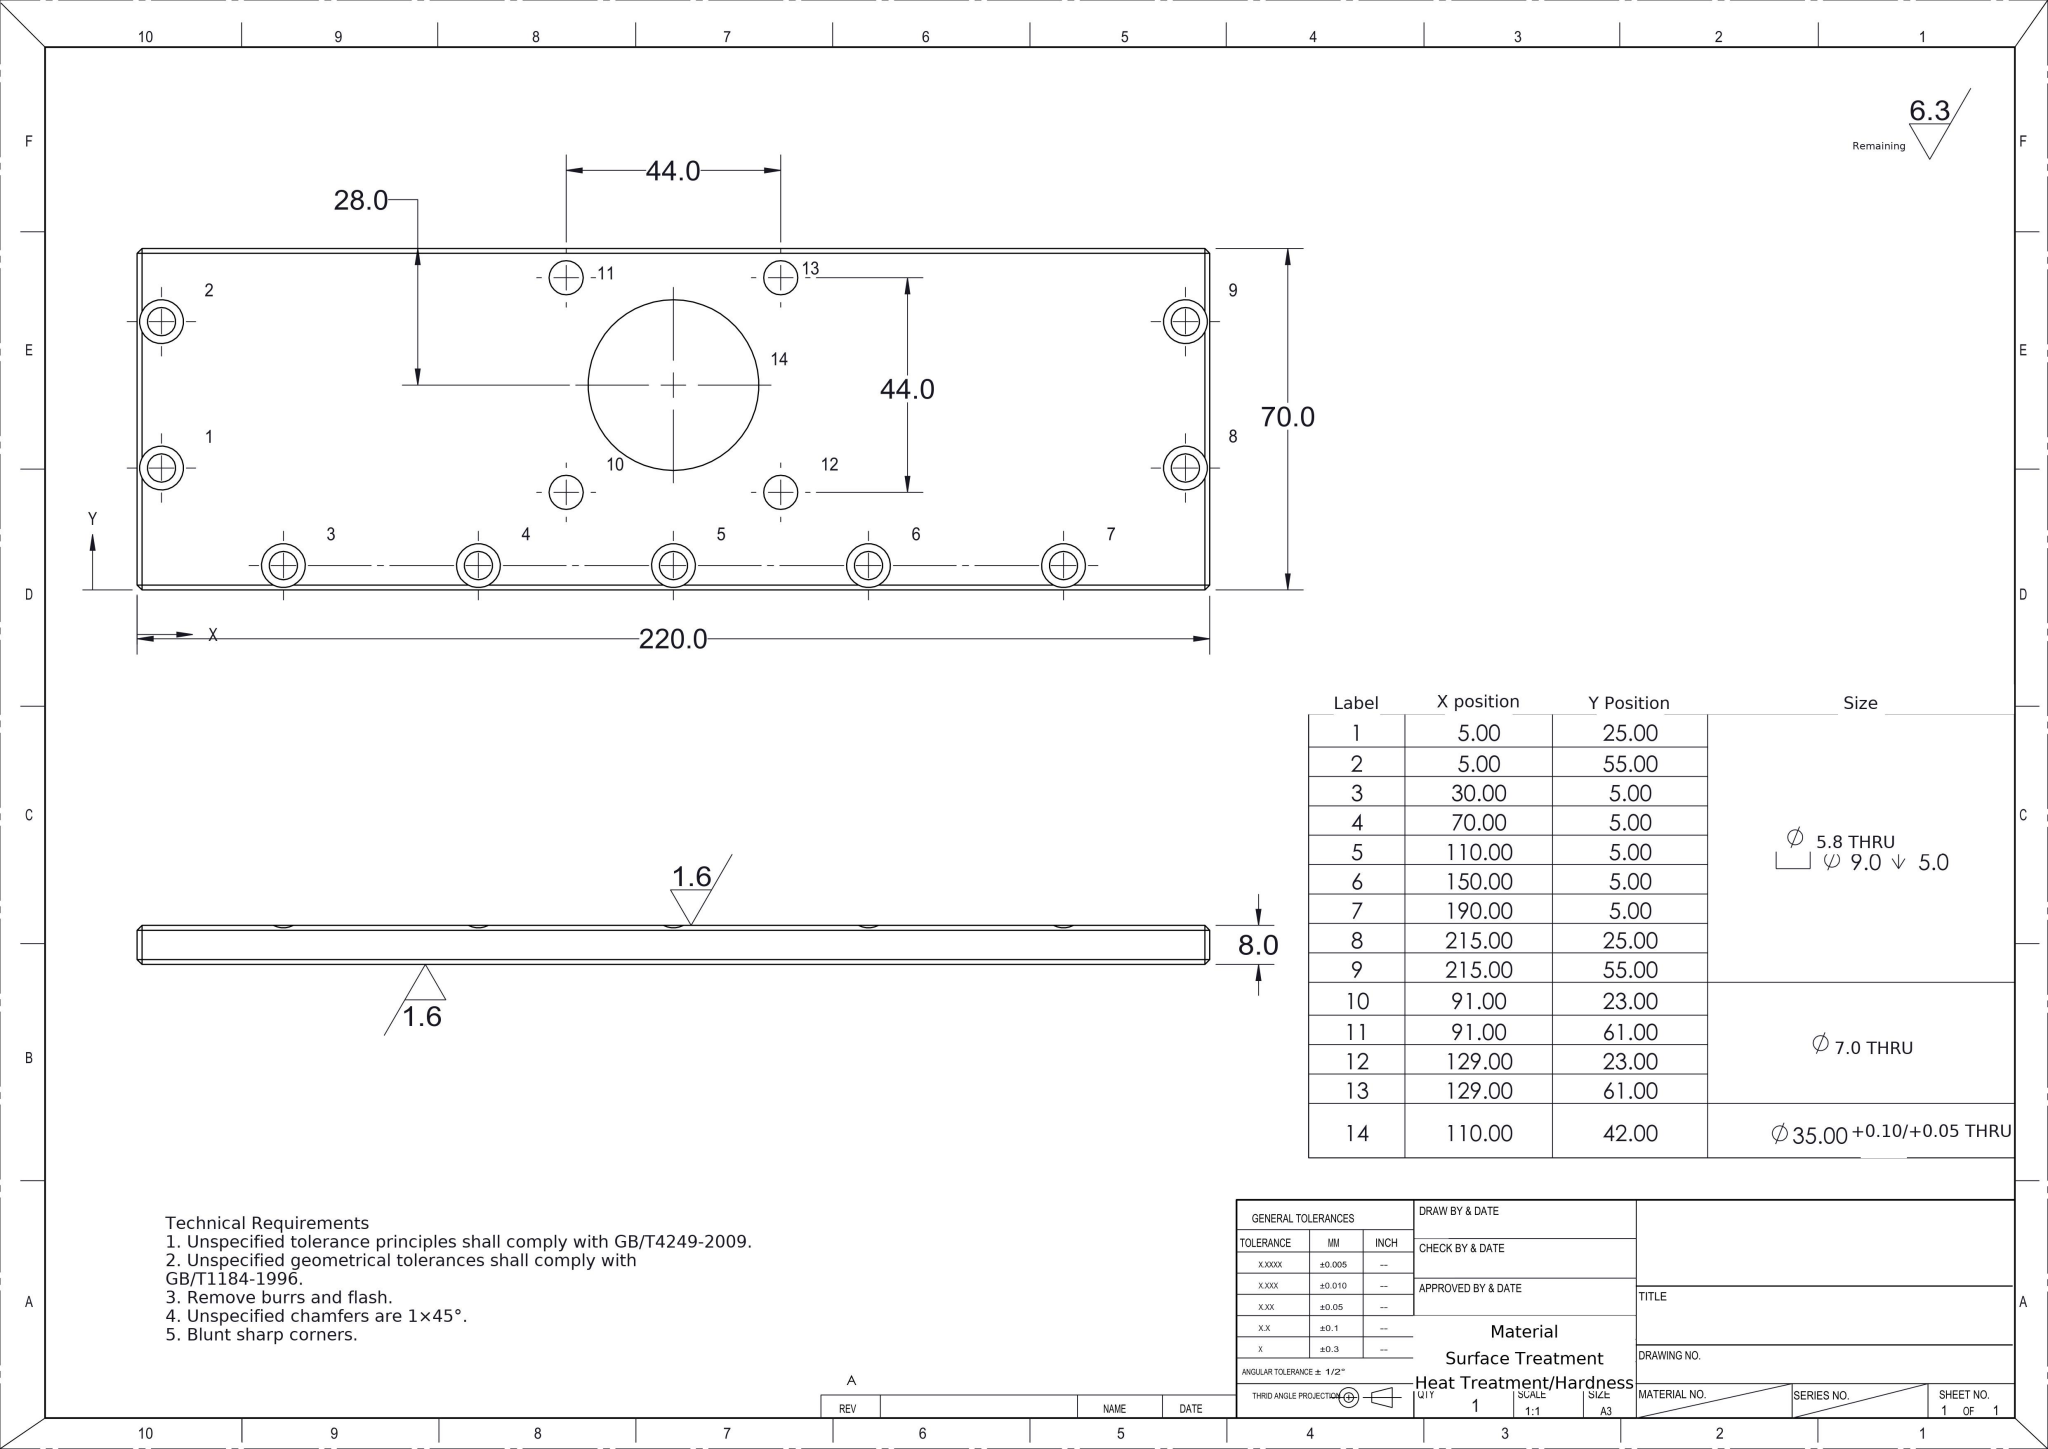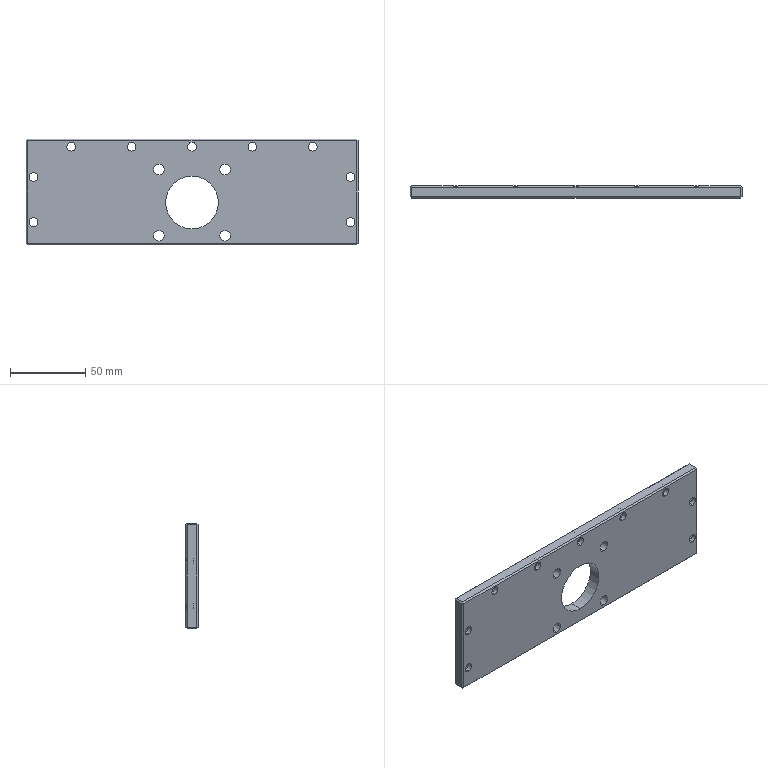Part | NX | mm | 1 solid | 81 faces | box 220 x 8 x 70 mm | volume 110107 mm3 | cylinder 46 | plane 35 | commonest cylinder face diameters 9 x18 5.8 x18 7 x8 35 x2